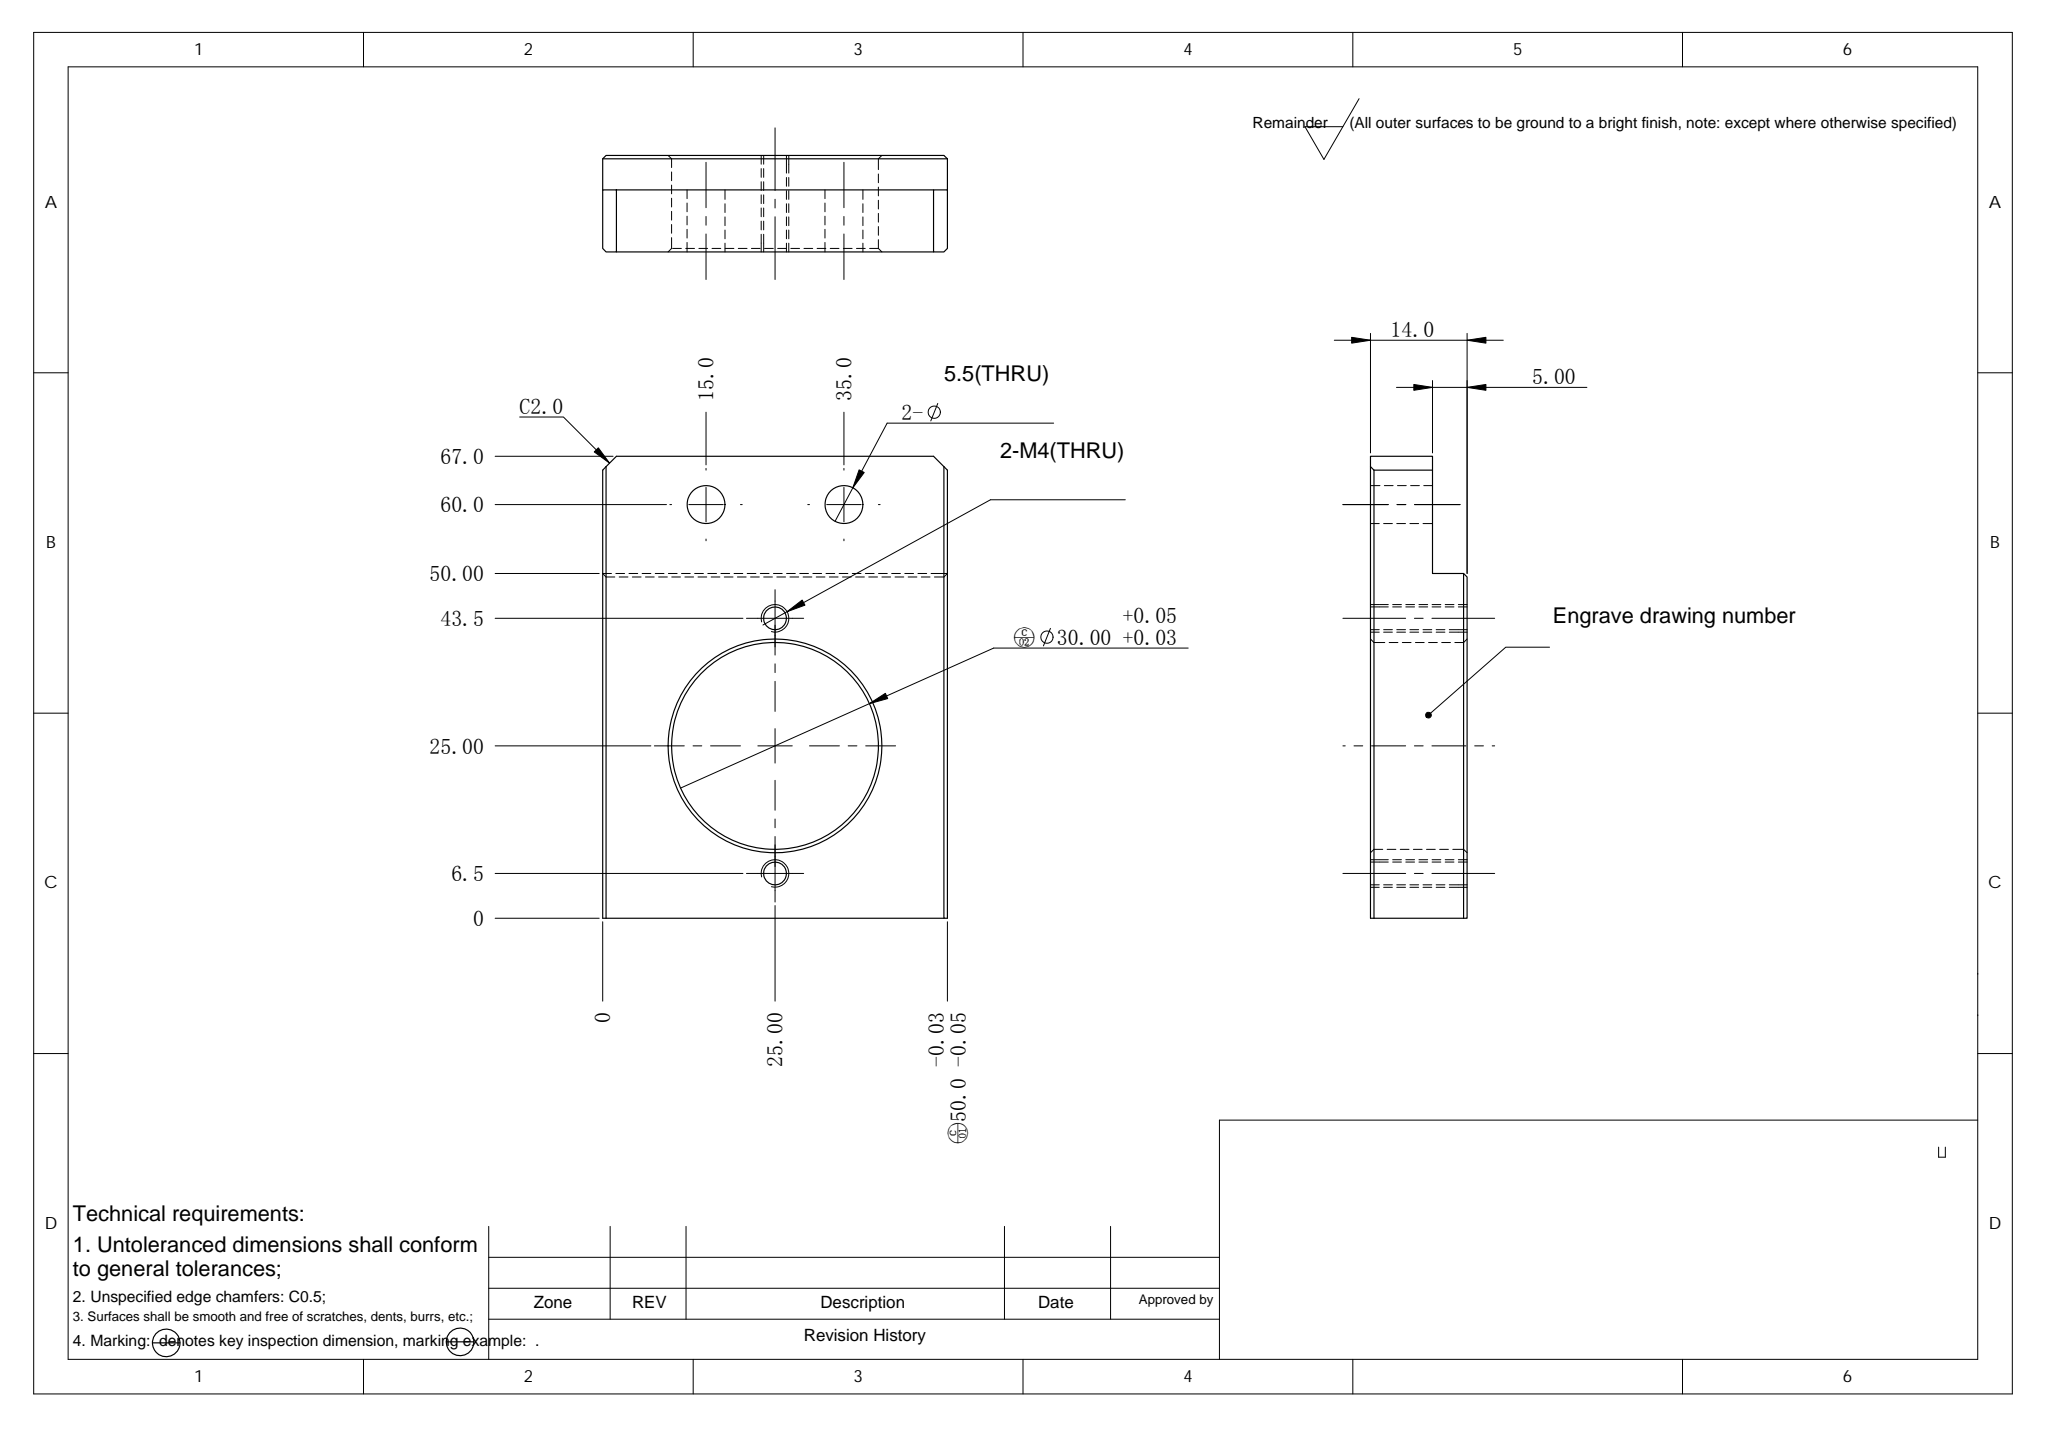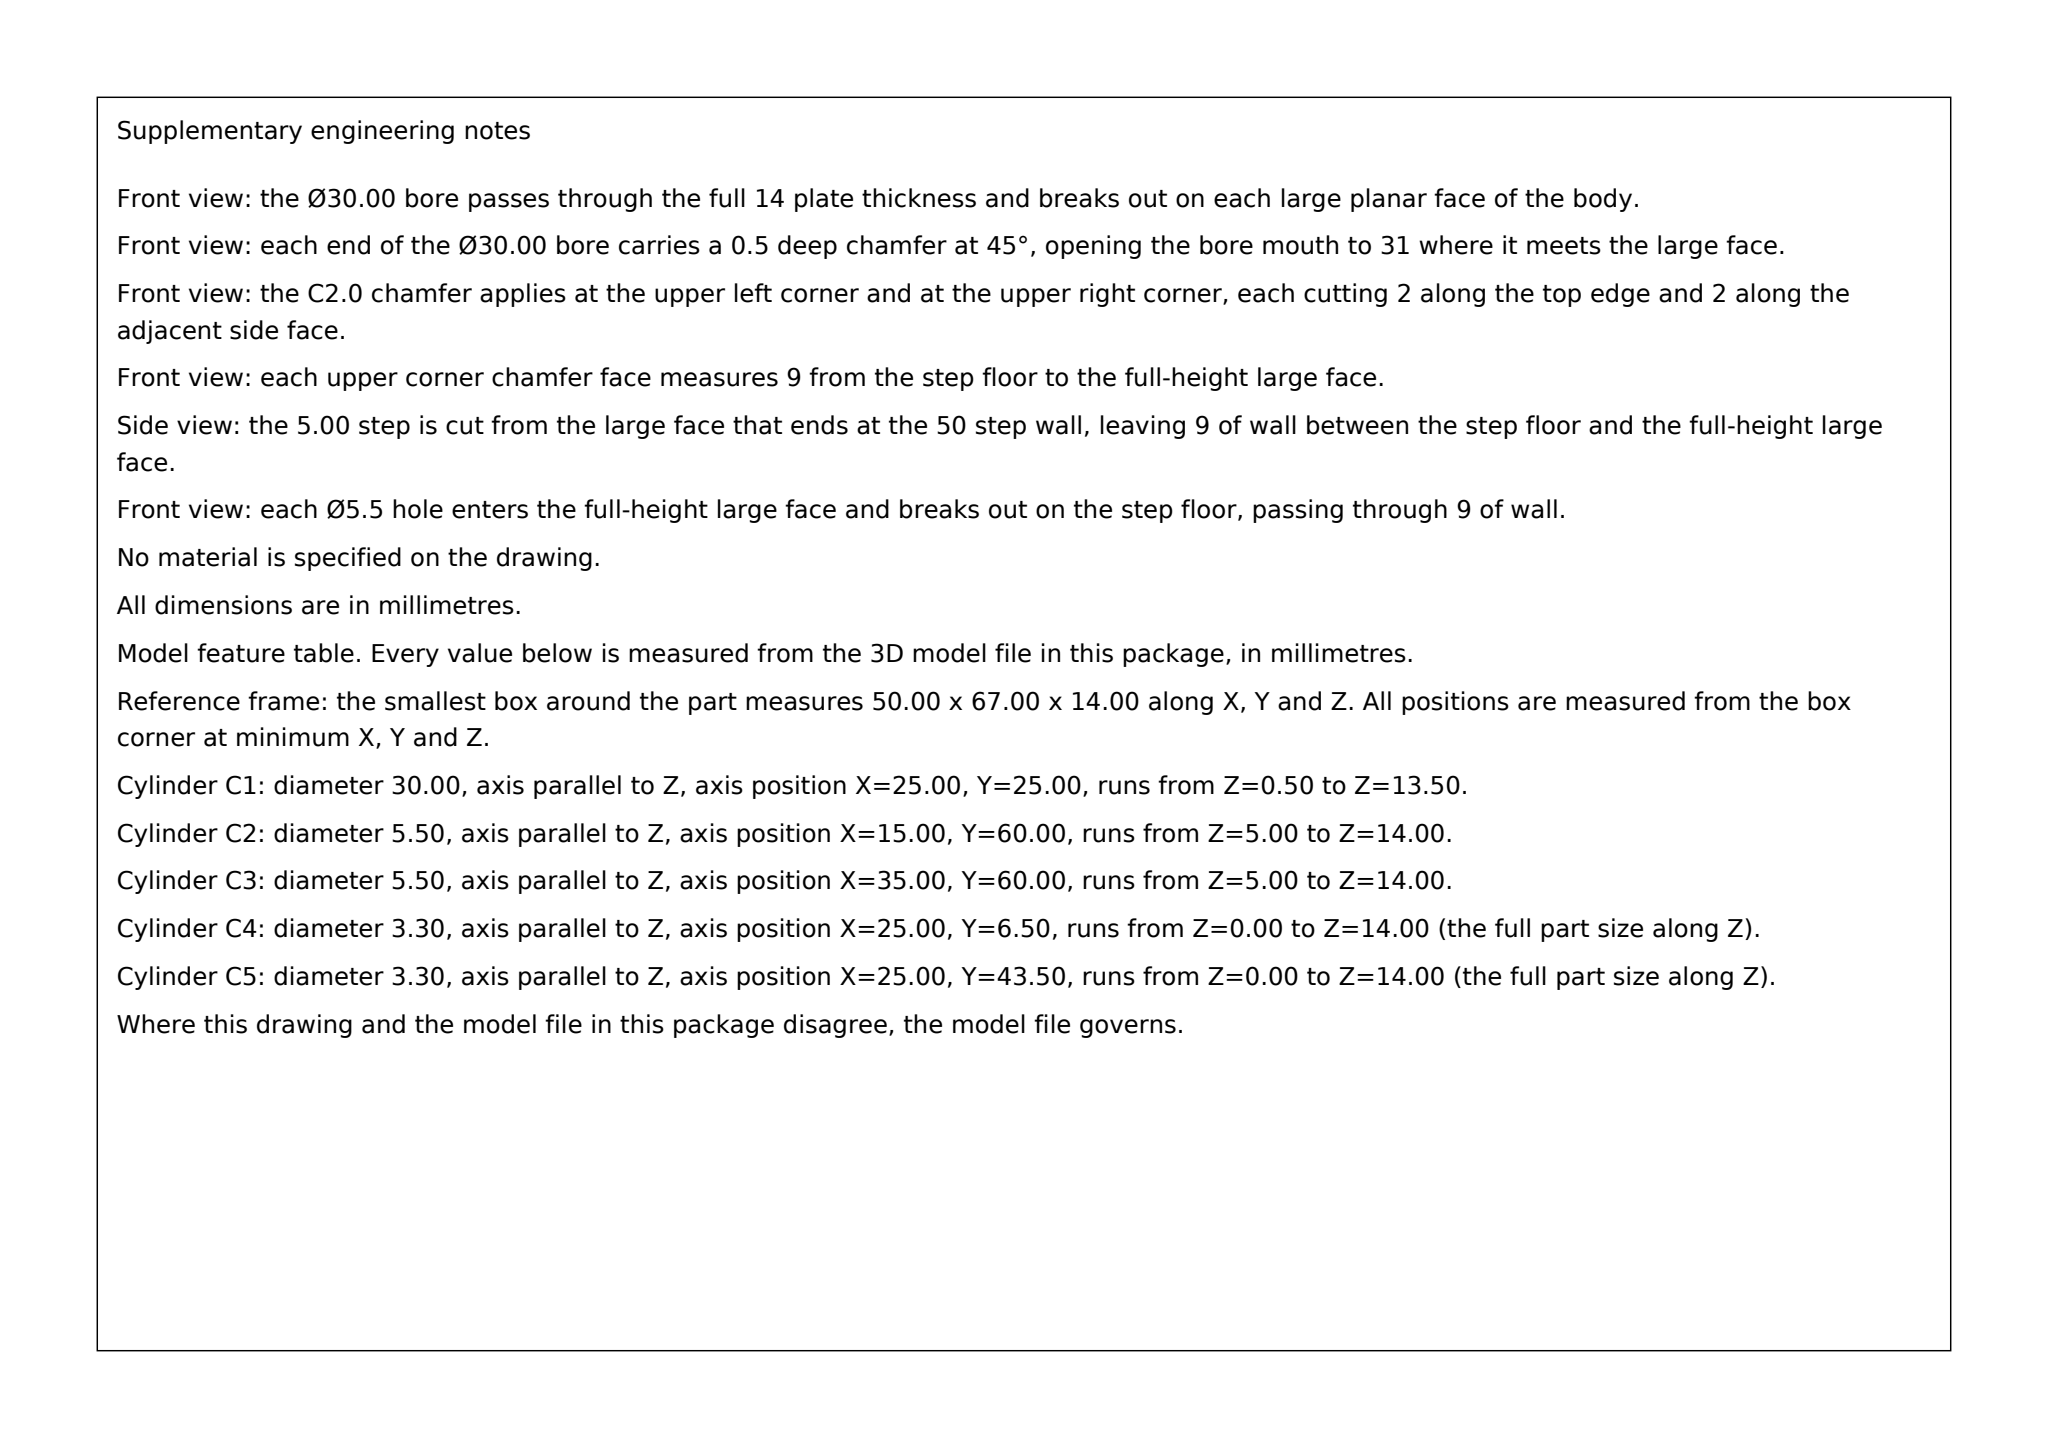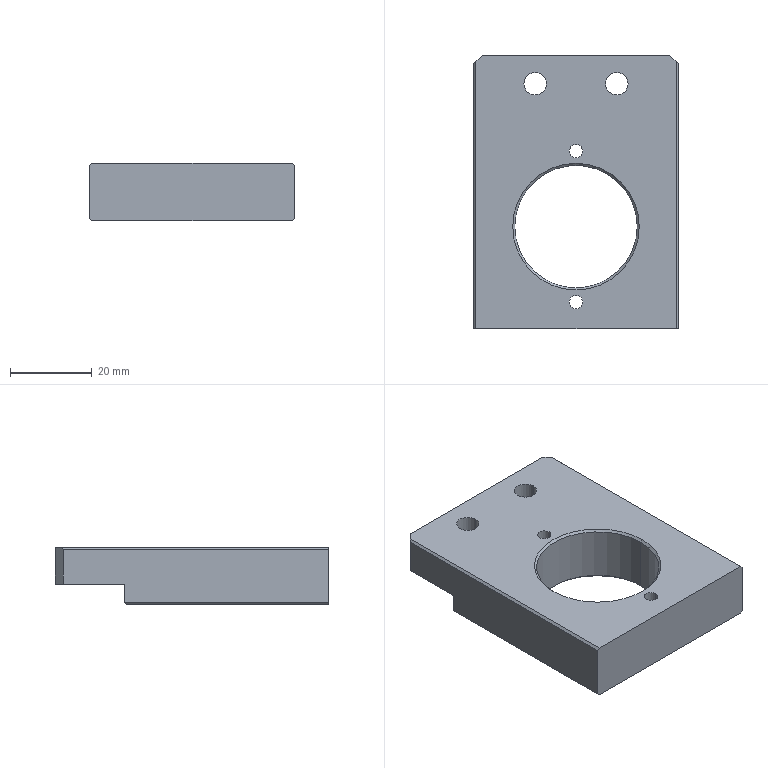Part | SolidWorks | mm | 1 solid | 29 faces | box 50 x 67 x 14 mm | volume 31992 mm3 | plane 15 | cylinder 10 | cone 4 | commonest cylinder face diameters 3.3 x4 5.5 x4 30 x2
Drawing notes:
STEP 17.0 WIDE (Y50.0-67.0) x FULL 50.0 x 5.00 DP | from the solid: z plane 5.0 step; y planes 50.0 and 67.0; x extent 0 to 50.0
Ø30.00 BORE THRU 14.0 THK | from the solid: Ø30 cyl L=13.0 + 0.5 chamfer each end = 14.0 = part thickness (z planes 0 and 14.0)
Ø30.00 BORE: C0.5 x 45° BOTH ENDS (TO Ø31.0) | from the solid: cones 90° incl, ref dia 30.0 to 31.0, qty 2 (one each end of bore)
2X C2.0 x 45° CHAMFER ON TOP CORNERS (AT Y=67.0, X=0 AND X=50.0), FULL DEPTH FROM Z=5.0 TO Z=14.0 | from the solid: inclined_planes: angle_to_xyz_axes [45,45,90] at bbox_from [0,65,5] and [48,65,5], size [2,2,9]
build123d program:
from build123d import *

# Parameters (mm, degrees)
SKETCH1_W                      = 50
SKETCH1_H                      = 70
BOSS_EXTRUDE1_DEPTH            = 14
SKETCH2_W                      = 5
SKETCH2_H                      = 20
CUT_EXTRUDE1_DEPTH             = 88.155
SKETCH3_R                      = 15
CUT_EXTRUDE2_DEPTH             = 88.155
F_5_5_5_5_DIAMETER_HOLE1_D     = 5.5
F_5_5_5_5_DIAMETER_HOLE1_DEPTH = 12
F_5_5_5_5_DIAMETER_HOLE1_TIP   = 1.652
M4_TAPPED_HOLE1_D              = 3.3
CHAMFER2_SIZE                  = 0.5
SKETCH8_W                      = 50
SKETCH8_H                      = 3
CUT_EXTRUDE3_DEPTH             = 88.155
CHAMFER3_SIZE                  = 2


with BuildPart() as part:
    # Sketch1 → Boss-Extrude1 (new body)
    with BuildSketch(Plane.XY):
        with Locations((25, 35)):
            Rectangle(SKETCH1_W, SKETCH1_H)
    extrude(amount=BOSS_EXTRUDE1_DEPTH)

    # Sketch2 → Cut-Extrude1 (cut, through all)
    with BuildSketch(Plane(origin=(50, 0, 0), x_dir=(0, 0, -1), z_dir=(1, 0, 0))):
        with Locations((-2.5, 60)):
            Rectangle(SKETCH2_W, SKETCH2_H)
    extrude(amount=-CUT_EXTRUDE1_DEPTH, mode=Mode.SUBTRACT)

    # Sketch3 → Cut-Extrude2 (cut, through all)
    with BuildSketch(Plane.XY.offset(14)):
        with Locations((25, 25)):
            Circle(SKETCH3_R)
    extrude(amount=-CUT_EXTRUDE2_DEPTH, mode=Mode.SUBTRACT)

    # 5.5 _5.5_ Diameter Hole1
    with Locations(Plane.XY.offset(14)):
        with Locations((15, 60), (35, 60)):
            Hole(F_5_5_5_5_DIAMETER_HOLE1_D / 2, depth=F_5_5_5_5_DIAMETER_HOLE1_DEPTH)
            with Locations((0, 0, -(F_5_5_5_5_DIAMETER_HOLE1_DEPTH + F_5_5_5_5_DIAMETER_HOLE1_TIP / 2))):  # 118° drill point
                Cone(0, F_5_5_5_5_DIAMETER_HOLE1_D / 2, F_5_5_5_5_DIAMETER_HOLE1_TIP, mode=Mode.SUBTRACT)

    # M4 Tapped Hole1 (through all)
    with Locations(Plane.XY.offset(14)):
        with Locations((25, 43.5), (25, 6.5)):
            Hole(M4_TAPPED_HOLE1_D / 2)

    # Chamfer2
    chamfer2_edges = [part.edges().sort_by_distance(p)[0] for p in [
        (50, 35, 14),
        (0, 25, 0),
        (25, 50, 0),
        (10, 25, 0),
        (10, 25, 14),
        (0, 35, 14),
        (50, 25, 0),
    ]]
    chamfer(chamfer2_edges, length=CHAMFER2_SIZE)

    # Sketch8 → Cut-Extrude3 (cut, through all)
    with BuildSketch(Plane.XY.offset(14)):
        with Locations((25, 68.5)):
            Rectangle(SKETCH8_W, SKETCH8_H)
    extrude(amount=-CUT_EXTRUDE3_DEPTH, mode=Mode.SUBTRACT)

    # Chamfer3
    chamfer3_edges = [part.edges().sort_by_distance(p)[0] for p in [
        (0, 67, 9.25),
        (50, 67, 9.25),
    ]]
    chamfer(chamfer3_edges, length=CHAMFER3_SIZE)


solid = part.part
STEP:
#1=CARTESIAN_POINT('',(10.,25.,13.5));
#2=VERTEX_POINT('',#1);
#3=CARTESIAN_POINT('',(40.,25.,13.5));
#4=VERTEX_POINT('',#3);
#5=CARTESIAN_POINT('',(25.,25.,13.5));
#6=DIRECTION('',(0.,0.,1.));
#7=DIRECTION('',(-1.,0.,0.));
#8=AXIS2_PLACEMENT_3D('',#5,#6,#7);
#9=CIRCLE('',#8,15.);
#10=EDGE_CURVE('',#2,#4,#9,.T.);
#11=ORIENTED_EDGE('',*,*,#10,.F.);
#12=CARTESIAN_POINT('',(9.5,25.,14.));
#13=VERTEX_POINT('',#12);
#14=CARTESIAN_POINT('',(10.,25.,13.5));
#15=DIRECTION('',(-0.7071,0.,0.7071));
#16=VECTOR('',#15,1000.);
#17=LINE('',#14,#16);
#18=EDGE_CURVE('',#2,#13,#17,.T.);
#19=ORIENTED_EDGE('',*,*,#18,.T.);
#20=CARTESIAN_POINT('',(40.5,25.,14.));
#21=VERTEX_POINT('',#20);
#22=CARTESIAN_POINT('',(25.,25.,14.));
#23=DIRECTION('',(0.,0.,-1.));
#24=DIRECTION('',(-1.,0.,0.));
#25=AXIS2_PLACEMENT_3D('',#22,#23,#24);
#26=CIRCLE('',#25,15.5);
#27=EDGE_CURVE('',#21,#13,#26,.T.);
#28=ORIENTED_EDGE('',*,*,#27,.F.);
#29=CARTESIAN_POINT('',(40.,25.,13.5));
#30=DIRECTION('',(0.7071,0.,0.7071));
#31=VECTOR('',#30,1000.);
#32=LINE('',#29,#31);
#33=EDGE_CURVE('',#4,#21,#32,.T.);
#34=ORIENTED_EDGE('',*,*,#33,.F.);
#35=EDGE_LOOP('',(#11,#19,#28,#34));
#36=FACE_OUTER_BOUND('',#35,.T.);
#37=CARTESIAN_POINT('',(25.,25.,13.5));
#38=DIRECTION('',(0.,0.,1.));
#39=DIRECTION('',(1.,0.,0.));
#40=AXIS2_PLACEMENT_3D('',#37,#38,#39);
#41=CONICAL_SURFACE('',#40,15.,0.7854);
#42=ADVANCED_FACE('',(#36),#41,.F.);
#43=CARTESIAN_POINT('',(40.,25.,0.5));
#44=VERTEX_POINT('',#43);
#45=CARTESIAN_POINT('',(10.,25.,0.5));
#46=VERTEX_POINT('',#45);
#47=CARTESIAN_POINT('',(25.,25.,0.5));
#48=DIRECTION('',(0.,0.,-1.));
#49=DIRECTION('',(-1.,0.,0.));
#50=AXIS2_PLACEMENT_3D('',#47,#48,#49);
#51=CIRCLE('',#50,15.);
#52=EDGE_CURVE('',#44,#46,#51,.T.);
#53=ORIENTED_EDGE('',*,*,#52,.F.);
#54=CARTESIAN_POINT('',(40.5,25.,0.));
#55=VERTEX_POINT('',#54);
#56=CARTESIAN_POINT('',(40.5,25.,0.));
#57=DIRECTION('',(0.7071,0.,-0.7071));
#58=VECTOR('',#57,1000.);
#59=LINE('',#56,#58);
#60=EDGE_CURVE('',#44,#55,#59,.T.);
#61=ORIENTED_EDGE('',*,*,#60,.T.);
#62=CARTESIAN_POINT('',(9.5,25.,0.));
#63=VERTEX_POINT('',#62);
#64=CARTESIAN_POINT('',(25.,25.,0.));
#65=DIRECTION('',(0.,0.,1.));
#66=DIRECTION('',(-1.,0.,0.));
#67=AXIS2_PLACEMENT_3D('',#64,#65,#66);
#68=CIRCLE('',#67,15.5);
#69=EDGE_CURVE('',#63,#55,#68,.T.);
#70=ORIENTED_EDGE('',*,*,#69,.F.);
#71=CARTESIAN_POINT('',(9.5,25.,0.));
#72=DIRECTION('',(-0.7071,0.,-0.7071));
#73=VECTOR('',#72,1000.);
#74=LINE('',#71,#73);
#75=EDGE_CURVE('',#46,#63,#74,.T.);
#76=ORIENTED_EDGE('',*,*,#75,.F.);
#77=EDGE_LOOP('',(#53,#61,#70,#76));
#78=FACE_OUTER_BOUND('',#77,.T.);
#79=CARTESIAN_POINT('',(25.,25.,0.));
#80=DIRECTION('',(0.,0.,-1.));
#81=DIRECTION('',(-1.,0.,0.));
#82=AXIS2_PLACEMENT_3D('',#79,#80,#81);
#83=CONICAL_SURFACE('',#82,15.5,0.7854);
#84=ADVANCED_FACE('',(#78),#83,.F.);
#85=CARTESIAN_POINT('',(23.35,43.5,-0.));
#86=VERTEX_POINT('',#85);
#87=CARTESIAN_POINT('',(26.65,43.5,-0.));
#88=VERTEX_POINT('',#87);
#89=CARTESIAN_POINT('',(25.,43.5,-0.));
#90=DIRECTION('',(0.,0.,1.));
#91=DIRECTION('',(1.,0.,0.));
#92=AXIS2_PLACEMENT_3D('',#89,#90,#91);
#93=CIRCLE('',#92,1.65);
#94=EDGE_CURVE('',#86,#88,#93,.T.);
#95=ORIENTED_EDGE('',*,*,#94,.F.);
#96=CARTESIAN_POINT('',(23.35,43.5,14.));
#97=VERTEX_POINT('',#96);
#98=CARTESIAN_POINT('',(23.35,43.5,14.));
#99=DIRECTION('',(0.,0.,1.));
#100=VECTOR('',#99,1000.);
#101=LINE('',#98,#100);
#102=EDGE_CURVE('',#86,#97,#101,.T.);
#103=ORIENTED_EDGE('',*,*,#102,.T.);
#104=CARTESIAN_POINT('',(26.65,43.5,14.));
#105=VERTEX_POINT('',#104);
#106=CARTESIAN_POINT('',(25.,43.5,14.));
#107=DIRECTION('',(0.,0.,1.));
#108=DIRECTION('',(1.,0.,0.));
#109=AXIS2_PLACEMENT_3D('',#106,#107,#108);
#110=CIRCLE('',#109,1.65);
#111=EDGE_CURVE('',#97,#105,#110,.T.);
#112=ORIENTED_EDGE('',*,*,#111,.T.);
#113=CARTESIAN_POINT('',(26.65,43.5,14.));
#114=DIRECTION('',(0.,0.,1.));
#115=VECTOR('',#114,1000.);
#116=LINE('',#113,#115);
#117=EDGE_CURVE('',#88,#105,#116,.T.);
#118=ORIENTED_EDGE('',*,*,#117,.F.);
#119=EDGE_LOOP('',(#95,#103,#112,#118));
#120=FACE_OUTER_BOUND('',#119,.T.);
#121=CARTESIAN_POINT('',(25.,43.5,14.));
#122=DIRECTION('',(0.,0.,1.));
#123=DIRECTION('',(1.,0.,0.));
#124=AXIS2_PLACEMENT_3D('',#121,#122,#123);
#125=CYLINDRICAL_SURFACE('',#124,1.65);
#126=ADVANCED_FACE('',(#120),#125,.F.);
#127=CARTESIAN_POINT('',(23.35,6.5,-0.));
#128=VERTEX_POINT('',#127);
#129=CARTESIAN_POINT('',(26.65,6.5,-0.));
#130=VERTEX_POINT('',#129);
#131=CARTESIAN_POINT('',(25.,6.5,-0.));
#132=DIRECTION('',(0.,0.,1.));
#133=DIRECTION('',(1.,0.,0.));
#134=AXIS2_PLACEMENT_3D('',#131,#132,#133);
#135=CIRCLE('',#134,1.65);
#136=EDGE_CURVE('',#128,#130,#135,.T.);
#137=ORIENTED_EDGE('',*,*,#136,.F.);
#138=CARTESIAN_POINT('',(23.35,6.5,14.));
#139=VERTEX_POINT('',#138);
#140=CARTESIAN_POINT('',(23.35,6.5,14.));
#141=DIRECTION('',(0.,0.,1.));
#142=VECTOR('',#141,1000.);
#143=LINE('',#140,#142);
#144=EDGE_CURVE('',#128,#139,#143,.T.);
#145=ORIENTED_EDGE('',*,*,#144,.T.);
#146=CARTESIAN_POINT('',(26.65,6.5,14.));
#147=VERTEX_POINT('',#146);
#148=CARTESIAN_POINT('',(25.,6.5,14.));
#149=DIRECTION('',(0.,0.,1.));
#150=DIRECTION('',(1.,0.,0.));
#151=AXIS2_PLACEMENT_3D('',#148,#149,#150);
#152=CIRCLE('',#151,1.65);
#153=EDGE_CURVE('',#139,#147,#152,.T.);
#154=ORIENTED_EDGE('',*,*,#153,.T.);
#155=CARTESIAN_POINT('',(26.65,6.5,14.));
#156=DIRECTION('',(0.,0.,1.));
#157=VECTOR('',#156,1000.);
#158=LINE('',#155,#157);
#159=EDGE_CURVE('',#130,#147,#158,.T.);
#160=ORIENTED_EDGE('',*,*,#159,.F.);
#161=EDGE_LOOP('',(#137,#145,#154,#160));
#162=FACE_OUTER_BOUND('',#161,.T.);
#163=CARTESIAN_POINT('',(25.,6.5,14.));
#164=DIRECTION('',(0.,0.,1.));
#165=DIRECTION('',(1.,0.,0.));
#166=AXIS2_PLACEMENT_3D('',#163,#164,#165);
#167=CYLINDRICAL_SURFACE('',#166,1.65);
#168=ADVANCED_FACE('',(#162),#167,.F.);
#169=CARTESIAN_POINT('',(12.25,60.,5.));
#170=VERTEX_POINT('',#169);
#171=CARTESIAN_POINT('',(17.75,60.,5.));
#172=VERTEX_POINT('',#171);
#173=CARTESIAN_POINT('',(15.,60.,5.));
#174=DIRECTION('',(0.,-0.,1.));
#175=DIRECTION('',(0.,-1.,0.));
#176=AXIS2_PLACEMENT_3D('',#173,#174,#175);
#177=CIRCLE('',#176,2.75);
#178=EDGE_CURVE('',#170,#172,#177,.T.);
#179=ORIENTED_EDGE('',*,*,#178,.F.);
#180=CARTESIAN_POINT('',(12.25,60.,14.));
#181=VERTEX_POINT('',#180);
#182=CARTESIAN_POINT('',(12.25,60.,14.));
#183=DIRECTION('',(0.,0.,1.));
#184=VECTOR('',#183,1000.);
#185=LINE('',#182,#184);
#186=EDGE_CURVE('',#170,#181,#185,.T.);
#187=ORIENTED_EDGE('',*,*,#186,.T.);
#188=CARTESIAN_POINT('',(17.75,60.,14.));
#189=VERTEX_POINT('',#188);
#190=CARTESIAN_POINT('',(15.,60.,14.));
#191=DIRECTION('',(0.,0.,1.));
#192=DIRECTION('',(1.,0.,0.));
#193=AXIS2_PLACEMENT_3D('',#190,#191,#192);
#194=CIRCLE('',#193,2.75);
#195=EDGE_CURVE('',#181,#189,#194,.T.);
#196=ORIENTED_EDGE('',*,*,#195,.T.);
#197=CARTESIAN_POINT('',(17.75,60.,14.));
#198=DIRECTION('',(0.,0.,1.));
#199=VECTOR('',#198,1000.);
#200=LINE('',#197,#199);
#201=EDGE_CURVE('',#172,#189,#200,.T.);
#202=ORIENTED_EDGE('',*,*,#201,.F.);
#203=EDGE_LOOP('',(#179,#187,#196,#202));
#204=FACE_OUTER_BOUND('',#203,.T.);
#205=CARTESIAN_POINT('',(15.,60.,14.));
#206=DIRECTION('',(0.,0.,1.));
#207=DIRECTION('',(1.,0.,0.));
#208=AXIS2_PLACEMENT_3D('',#205,#206,#207);
#209=CYLINDRICAL_SURFACE('',#208,2.75);
#210=ADVANCED_FACE('',(#204),#209,.F.);
#211=CARTESIAN_POINT('',(32.25,60.,5.));
#212=VERTEX_POINT('',#211);
#213=CARTESIAN_POINT('',(37.75,60.,5.));
#214=VERTEX_POINT('',#213);
#215=CARTESIAN_POINT('',(35.,60.,5.));
#216=DIRECTION('',(0.,-0.,1.));
#217=DIRECTION('',(0.,-1.,0.));
#218=AXIS2_PLACEMENT_3D('',#215,#216,#217);
#219=CIRCLE('',#218,2.75);
#220=EDGE_CURVE('',#212,#214,#219,.T.);
#221=ORIENTED_EDGE('',*,*,#220,.F.);
#222=CARTESIAN_POINT('',(32.25,60.,14.));
#223=VERTEX_POINT('',#222);
#224=CARTESIAN_POINT('',(32.25,60.,14.));
#225=DIRECTION('',(0.,0.,1.));
#226=VECTOR('',#225,1000.);
#227=LINE('',#224,#226);
#228=EDGE_CURVE('',#212,#223,#227,.T.);
#229=ORIENTED_EDGE('',*,*,#228,.T.);
#230=CARTESIAN_POINT('',(37.75,60.,14.));
#231=VERTEX_POINT('',#230);
#232=CARTESIAN_POINT('',(35.,60.,14.));
#233=DIRECTION('',(0.,0.,1.));
#234=DIRECTION('',(1.,0.,0.));
#235=AXIS2_PLACEMENT_3D('',#232,#233,#234);
#236=CIRCLE('',#235,2.75);
#237=EDGE_CURVE('',#223,#231,#236,.T.);
#238=ORIENTED_EDGE('',*,*,#237,.T.);
#239=CARTESIAN_POINT('',(37.75,60.,14.));
#240=DIRECTION('',(0.,0.,1.));
#241=VECTOR('',#240,1000.);
#242=LINE('',#239,#241);
#243=EDGE_CURVE('',#214,#231,#242,.T.);
#244=ORIENTED_EDGE('',*,*,#243,.F.);
#245=EDGE_LOOP('',(#221,#229,#238,#244));
#246=FACE_OUTER_BOUND('',#245,.T.);
#247=CARTESIAN_POINT('',(35.,60.,14.));
#248=DIRECTION('',(0.,0.,1.));
#249=DIRECTION('',(1.,0.,0.));
#250=AXIS2_PLACEMENT_3D('',#247,#248,#249);
#251=CYLINDRICAL_SURFACE('',#250,2.75);
#252=ADVANCED_FACE('',(#246),#251,.F.);
#253=ORIENTED_EDGE('',*,*,#52,.T.);
#254=CARTESIAN_POINT('',(10.,25.,-0.));
#255=DIRECTION('',(0.,0.,1.));
#256=VECTOR('',#255,1000.);
#257=LINE('',#254,#256);
#258=EDGE_CURVE('',#46,#2,#257,.T.);
#259=ORIENTED_EDGE('',*,*,#258,.T.);
#260=ORIENTED_EDGE('',*,*,#10,.T.);
#261=CARTESIAN_POINT('',(40.,25.,-0.));
#262=DIRECTION('',(0.,0.,1.));
#263=VECTOR('',#262,1000.);
#264=LINE('',#261,#263);
#265=EDGE_CURVE('',#44,#4,#264,.T.);
#266=ORIENTED_EDGE('',*,*,#265,.F.);
#267=EDGE_LOOP('',(#253,#259,#260,#266));
#268=FACE_OUTER_BOUND('',#267,.T.);
#269=CARTESIAN_POINT('',(25.,25.,-0.));
#270=DIRECTION('',(0.,0.,1.));
#271=DIRECTION('',(1.,0.,0.));
#272=AXIS2_PLACEMENT_3D('',#269,#270,#271);
#273=CYLINDRICAL_SURFACE('',#272,15.);
#274=ADVANCED_FACE('',(#268),#273,.F.);
#275=CARTESIAN_POINT('',(0.,0.,13.5));
#276=VERTEX_POINT('',#275);
#277=CARTESIAN_POINT('',(0.,65.,13.5));
#278=VERTEX_POINT('',#277);
#279=CARTESIAN_POINT('',(0.,0.,13.5));
#280=DIRECTION('',(0.,1.,0.));
#281=VECTOR('',#280,1000.);
#282=LINE('',#279,#281);
#283=EDGE_CURVE('',#276,#278,#282,.T.);
#284=ORIENTED_EDGE('',*,*,#283,.T.);
#285=CARTESIAN_POINT('',(-0.,65.,5.));
#286=VERTEX_POINT('',#285);
#287=CARTESIAN_POINT('',(0.,65.,14.));
#288=DIRECTION('',(0.,0.,-1.));
#289=VECTOR('',#288,1000.);
#290=LINE('',#287,#289);
#291=EDGE_CURVE('',#278,#286,#290,.T.);
#292=ORIENTED_EDGE('',*,*,#291,.T.);
#293=CARTESIAN_POINT('',(0.,50.,5.));
#294=VERTEX_POINT('',#293);
#295=CARTESIAN_POINT('',(0.,70.,5.));
#296=DIRECTION('',(0.,-1.,-0.));
#297=VECTOR('',#296,1000.);
#298=LINE('',#295,#297);
#299=EDGE_CURVE('',#286,#294,#298,.T.);
#300=ORIENTED_EDGE('',*,*,#299,.T.);
#301=CARTESIAN_POINT('',(0.,50.,0.5));
#302=VERTEX_POINT('',#301);
#303=CARTESIAN_POINT('',(0.,50.,-0.));
#304=DIRECTION('',(0.,0.,-1.));
#305=VECTOR('',#304,1000.);
#306=LINE('',#303,#305);
#307=EDGE_CURVE('',#294,#302,#306,.T.);
#308=ORIENTED_EDGE('',*,*,#307,.T.);
#309=CARTESIAN_POINT('',(-0.,0.,0.5));
#310=VERTEX_POINT('',#309);
#311=CARTESIAN_POINT('',(0.,0.,0.5));
#312=DIRECTION('',(0.,-1.,0.));
#313=VECTOR('',#312,1000.);
#314=LINE('',#311,#313);
#315=EDGE_CURVE('',#302,#310,#314,.T.);
#316=ORIENTED_EDGE('',*,*,#315,.T.);
#317=CARTESIAN_POINT('',(0.,0.,14.));
#318=DIRECTION('',(0.,0.,-1.));
#319=VECTOR('',#318,1000.);
#320=LINE('',#317,#319);
#321=EDGE_CURVE('',#276,#310,#320,.T.);
#322=ORIENTED_EDGE('',*,*,#321,.F.);
#323=EDGE_LOOP('',(#284,#292,#300,#308,#316,#322));
#324=FACE_OUTER_BOUND('',#323,.T.);
#325=CARTESIAN_POINT('',(0.,0.,14.));
#326=DIRECTION('',(1.,0.,0.));
#327=DIRECTION('',(0.,0.,-1.));
#328=AXIS2_PLACEMENT_3D('',#325,#326,#327);
#329=PLANE('',#328);
#330=ADVANCED_FACE('',(#324),#329,.F.);
#331=CARTESIAN_POINT('',(0.5,0.,14.));
#332=VERTEX_POINT('',#331);
#333=CARTESIAN_POINT('',(49.5,0.,14.));
#334=VERTEX_POINT('',#333);
#335=CARTESIAN_POINT('',(0.,0.,14.));
#336=DIRECTION('',(1.,0.,0.));
#337=VECTOR('',#336,1000.);
#338=LINE('',#335,#337);
#339=EDGE_CURVE('',#332,#334,#338,.T.);
#340=ORIENTED_EDGE('',*,*,#339,.F.);
#341=CARTESIAN_POINT('',(0.5,0.,14.));
#342=DIRECTION('',(-0.7071,0.,-0.7071));
#343=VECTOR('',#342,1000.);
#344=LINE('',#341,#343);
#345=EDGE_CURVE('',#332,#276,#344,.T.);
#346=ORIENTED_EDGE('',*,*,#345,.T.);
#347=ORIENTED_EDGE('',*,*,#321,.T.);
#348=CARTESIAN_POINT('',(0.5,0.,0.));
#349=VERTEX_POINT('',#348);
#350=CARTESIAN_POINT('',(0.,0.,0.5));
#351=DIRECTION('',(0.7071,0.,-0.7071));
#352=VECTOR('',#351,1000.);
#353=LINE('',#350,#352);
#354=EDGE_CURVE('',#310,#349,#353,.T.);
#355=ORIENTED_EDGE('',*,*,#354,.T.);
#356=CARTESIAN_POINT('',(49.5,0.,-0.));
#357=VERTEX_POINT('',#356);
#358=CARTESIAN_POINT('',(0.,0.,0.));
#359=DIRECTION('',(1.,0.,0.));
#360=VECTOR('',#359,1000.);
#361=LINE('',#358,#360);
#362=EDGE_CURVE('',#349,#357,#361,.T.);
#363=ORIENTED_EDGE('',*,*,#362,.T.);
#364=CARTESIAN_POINT('',(50.,0.,0.5));
#365=VERTEX_POINT('',#364);
#366=CARTESIAN_POINT('',(50.,0.,0.5));
#367=DIRECTION('',(0.7071,0.,0.7071));
#368=VECTOR('',#367,1000.);
#369=LINE('',#366,#368);
#370=EDGE_CURVE('',#357,#365,#369,.T.);
#371=ORIENTED_EDGE('',*,*,#370,.T.);
#372=CARTESIAN_POINT('',(50.,0.,13.5));
#373=VERTEX_POINT('',#372);
#374=CARTESIAN_POINT('',(50.,0.,14.));
#375=DIRECTION('',(0.,0.,-1.));
#376=VECTOR('',#375,1000.);
#377=LINE('',#374,#376);
#378=EDGE_CURVE('',#373,#365,#377,.T.);
#379=ORIENTED_EDGE('',*,*,#378,.F.);
#380=CARTESIAN_POINT('',(49.5,0.,14.));
#381=DIRECTION('',(-0.7071,0.,0.7071));
#382=VECTOR('',#381,1000.);
#383=LINE('',#380,#382);
#384=EDGE_CURVE('',#373,#334,#383,.T.);
#385=ORIENTED_EDGE('',*,*,#384,.T.);
#386=EDGE_LOOP('',(#340,#346,#347,#355,#363,#371,#379,#385));
#387=FACE_OUTER_BOUND('',#386,.T.);
#388=CARTESIAN_POINT('',(0.,0.,14.));
#389=DIRECTION('',(0.,1.,0.));
#390=DIRECTION('',(0.,0.,1.));
#391=AXIS2_PLACEMENT_3D('',#388,#389,#390);
#392=PLANE('',#391);
#393=ADVANCED_FACE('',(#387),#392,.F.);
#394=CARTESIAN_POINT('',(50.,65.,5.));
#395=VERTEX_POINT('',#394);
#396=CARTESIAN_POINT('',(50.,50.,5.));
#397=VERTEX_POINT('',#396);
#398=CARTESIAN_POINT('',(50.,70.,5.));
#399=DIRECTION('',(0.,-1.,-0.));
#400=VECTOR('',#399,1000.);
#401=LINE('',#398,#400);
#402=EDGE_CURVE('',#395,#397,#401,.T.);
#403=ORIENTED_EDGE('',*,*,#402,.F.);
#404=CARTESIAN_POINT('',(50.,65.,13.5));
#405=VERTEX_POINT('',#404);
#406=CARTESIAN_POINT('',(50.,65.,14.));
#407=DIRECTION('',(0.,0.,1.));
#408=VECTOR('',#407,1000.);
#409=LINE('',#406,#408);
#410=EDGE_CURVE('',#395,#405,#409,.T.);
#411=ORIENTED_EDGE('',*,*,#410,.T.);
#412=CARTESIAN_POINT('',(50.,0.,13.5));
#413=DIRECTION('',(0.,-1.,0.));
#414=VECTOR('',#413,1000.);
#415=LINE('',#412,#414);
#416=EDGE_CURVE('',#405,#373,#415,.T.);
#417=ORIENTED_EDGE('',*,*,#416,.T.);
#418=ORIENTED_EDGE('',*,*,#378,.T.);
#419=CARTESIAN_POINT('',(50.,50.,0.5));
#420=VERTEX_POINT('',#419);
#421=CARTESIAN_POINT('',(50.,50.,0.5));
#422=DIRECTION('',(0.,1.,0.));
#423=VECTOR('',#422,1000.);
#424=LINE('',#421,#423);
#425=EDGE_CURVE('',#365,#420,#424,.T.);
#426=ORIENTED_EDGE('',*,*,#425,.T.);
#427=CARTESIAN_POINT('',(50.,50.,-0.));
#428=DIRECTION('',(0.,0.,-1.));
#429=VECTOR('',#428,1000.);
#430=LINE('',#427,#429);
#431=EDGE_CURVE('',#397,#420,#430,.T.);
#432=ORIENTED_EDGE('',*,*,#431,.F.);
#433=EDGE_LOOP('',(#403,#411,#417,#418,#426,#432));
#434=FACE_OUTER_BOUND('',#433,.T.);
#435=CARTESIAN_POINT('',(50.,0.,14.));
#436=DIRECTION('',(-1.,0.,0.));
#437=DIRECTION('',(0.,0.,1.));
#438=AXIS2_PLACEMENT_3D('',#435,#436,#437);
#439=PLANE('',#438);
#440=ADVANCED_FACE('',(#434),#439,.F.);
#441=ORIENTED_EDGE('',*,*,#27,.T.);
#442=CARTESIAN_POINT('',(25.,25.,14.));
#443=DIRECTION('',(0.,0.,-1.));
#444=DIRECTION('',(-1.,0.,0.));
#445=AXIS2_PLACEMENT_3D('',#442,#443,#444);
#446=CIRCLE('',#445,15.5);
#447=EDGE_CURVE('',#13,#21,#446,.T.);
#448=ORIENTED_EDGE('',*,*,#447,.T.);
#449=EDGE_LOOP('',(#441,#448));
#450=FACE_BOUND('',#449,.T.);
#451=CARTESIAN_POINT('',(25.,43.5,14.));
#452=DIRECTION('',(0.,0.,1.));
#453=DIRECTION('',(1.,0.,0.));
#454=AXIS2_PLACEMENT_3D('',#451,#452,#453);
#455=CIRCLE('',#454,1.65);
#456=EDGE_CURVE('',#105,#97,#455,.T.);
#457=ORIENTED_EDGE('',*,*,#456,.F.);
#458=ORIENTED_EDGE('',*,*,#111,.F.);
#459=EDGE_LOOP('',(#457,#458));
#460=FACE_BOUND('',#459,.T.);
#461=CARTESIAN_POINT('',(25.,6.5,14.));
#462=DIRECTION('',(0.,0.,1.));
#463=DIRECTION('',(1.,0.,0.));
#464=AXIS2_PLACEMENT_3D('',#461,#462,#463);
#465=CIRCLE('',#464,1.65);
#466=EDGE_CURVE('',#147,#139,#465,.T.);
#467=ORIENTED_EDGE('',*,*,#466,.F.);
#468=ORIENTED_EDGE('',*,*,#153,.F.);
#469=EDGE_LOOP('',(#467,#468));
#470=FACE_BOUND('',#469,.T.);
#471=CARTESIAN_POINT('',(15.,60.,14.));
#472=DIRECTION('',(0.,0.,1.));
#473=DIRECTION('',(1.,0.,0.));
#474=AXIS2_PLACEMENT_3D('',#471,#472,#473);
#475=CIRCLE('',#474,2.75);
#476=EDGE_CURVE('',#189,#181,#475,.T.);
#477=ORIENTED_EDGE('',*,*,#476,.F.);
#478=ORIENTED_EDGE('',*,*,#195,.F.);
#479=EDGE_LOOP('',(#477,#478));
#480=FACE_BOUND('',#479,.T.);
#481=CARTESIAN_POINT('',(35.,60.,14.));
#482=DIRECTION('',(0.,0.,1.));
#483=DIRECTION('',(1.,0.,0.));
#484=AXIS2_PLACEMENT_3D('',#481,#482,#483);
#485=CIRCLE('',#484,2.75);
#486=EDGE_CURVE('',#231,#223,#485,.T.);
#487=ORIENTED_EDGE('',*,*,#486,.F.);
#488=ORIENTED_EDGE('',*,*,#237,.F.);
#489=EDGE_LOOP('',(#487,#488));
#490=FACE_BOUND('',#489,.T.);
#491=CARTESIAN_POINT('',(2.,67.,14.));
#492=VERTEX_POINT('',#491);
#493=CARTESIAN_POINT('',(48.,67.,14.));
#494=VERTEX_POINT('',#493);
#495=CARTESIAN_POINT('',(0.,67.,14.));
#496=DIRECTION('',(1.,0.,0.));
#497=VECTOR('',#496,1000.);
#498=LINE('',#495,#497);
#499=EDGE_CURVE('',#492,#494,#498,.T.);
#500=ORIENTED_EDGE('',*,*,#499,.F.);
#501=CARTESIAN_POINT('',(0.5,65.5,14.));
#502=VERTEX_POINT('',#501);
#503=CARTESIAN_POINT('',(2.,67.,14.));
#504=DIRECTION('',(-0.7071,-0.7071,0.));
#505=VECTOR('',#504,1000.);
#506=LINE('',#503,#505);
#507=EDGE_CURVE('',#492,#502,#506,.T.);
#508=ORIENTED_EDGE('',*,*,#507,.T.);
#509=CARTESIAN_POINT('',(0.5,0.,14.));
#510=DIRECTION('',(0.,-1.,0.));
#511=VECTOR('',#510,1000.);
#512=LINE('',#509,#511);
#513=EDGE_CURVE('',#502,#332,#512,.T.);
#514=ORIENTED_EDGE('',*,*,#513,.T.);
#515=ORIENTED_EDGE('',*,*,#339,.T.);
#516=CARTESIAN_POINT('',(49.5,65.5,14.));
#517=VERTEX_POINT('',#516);
#518=CARTESIAN_POINT('',(49.5,0.,14.));
#519=DIRECTION('',(0.,1.,0.));
#520=VECTOR('',#519,1000.);
#521=LINE('',#518,#520);
#522=EDGE_CURVE('',#334,#517,#521,.T.);
#523=ORIENTED_EDGE('',*,*,#522,.T.);
#524=CARTESIAN_POINT('',(50.,65.,14.));
#525=DIRECTION('',(-0.7071,0.7071,0.));
#526=VECTOR('',#525,1000.);
#527=LINE('',#524,#526);
#528=EDGE_CURVE('',#517,#494,#527,.T.);
#529=ORIENTED_EDGE('',*,*,#528,.T.);
#530=EDGE_LOOP('',(#500,#508,#514,#515,#523,#529));
#531=FACE_OUTER_BOUND('',#530,.T.);
#532=CARTESIAN_POINT('',(0.,0.,14.));
#533=DIRECTION('',(0.,0.,-1.));
#534=DIRECTION('',(-1.,0.,0.));
#535=AXIS2_PLACEMENT_3D('',#532,#533,#534);
#536=PLANE('',#535);
#537=ADVANCED_FACE('',(#450,#460,#470,#480,#490,#531),#536,.F.);
#538=ORIENTED_EDGE('',*,*,#69,.T.);
#539=CARTESIAN_POINT('',(25.,25.,0.));
#540=DIRECTION('',(0.,0.,1.));
#541=DIRECTION('',(-1.,0.,0.));
#542=AXIS2_PLACEMENT_3D('',#539,#540,#541);
#543=CIRCLE('',#542,15.5);
#544=EDGE_CURVE('',#55,#63,#543,.T.);
#545=ORIENTED_EDGE('',*,*,#544,.T.);
#546=EDGE_LOOP('',(#538,#545));
#547=FACE_BOUND('',#546,.T.);
#548=CARTESIAN_POINT('',(25.,43.5,-0.));
#549=DIRECTION('',(0.,0.,1.));
#550=DIRECTION('',(1.,0.,0.));
#551=AXIS2_PLACEMENT_3D('',#548,#549,#550);
#552=CIRCLE('',#551,1.65);
#553=EDGE_CURVE('',#88,#86,#552,.T.);
#554=ORIENTED_EDGE('',*,*,#553,.T.);
#555=ORIENTED_EDGE('',*,*,#94,.T.);
#556=EDGE_LOOP('',(#554,#555));
#557=FACE_BOUND('',#556,.T.);
#558=CARTESIAN_POINT('',(25.,6.5,-0.));
#559=DIRECTION('',(0.,0.,1.));
#560=DIRECTION('',(1.,0.,0.));
#561=AXIS2_PLACEMENT_3D('',#558,#559,#560);
#562=CIRCLE('',#561,1.65);
#563=EDGE_CURVE('',#130,#128,#562,.T.);
#564=ORIENTED_EDGE('',*,*,#563,.T.);
#565=ORIENTED_EDGE('',*,*,#136,.T.);
#566=EDGE_LOOP('',(#564,#565));
#567=FACE_BOUND('',#566,.T.);
#568=ORIENTED_EDGE('',*,*,#362,.F.);
#569=CARTESIAN_POINT('',(0.5,49.5,0.));
#570=VERTEX_POINT('',#569);
#571=CARTESIAN_POINT('',(0.5,50.,0.));
#572=DIRECTION('',(0.,1.,0.));
#573=VECTOR('',#572,1000.);
#574=LINE('',#571,#573);
#575=EDGE_CURVE('',#349,#570,#574,.T.);
#576=ORIENTED_EDGE('',*,*,#575,.T.);
#577=CARTESIAN_POINT('',(49.5,49.5,0.));
#578=VERTEX_POINT('',#577);
#579=CARTESIAN_POINT('',(50.,49.5,0.));
#580=DIRECTION('',(1.,0.,0.));
#581=VECTOR('',#580,1000.);
#582=LINE('',#579,#581);
#583=EDGE_CURVE('',#570,#578,#582,.T.);
#584=ORIENTED_EDGE('',*,*,#583,.T.);
#585=CARTESIAN_POINT('',(49.5,0.,0.));
#586=DIRECTION('',(0.,-1.,0.));
#587=VECTOR('',#586,1000.);
#588=LINE('',#585,#587);
#589=EDGE_CURVE('',#578,#357,#588,.T.);
#590=ORIENTED_EDGE('',*,*,#589,.T.);
#591=EDGE_LOOP('',(#568,#576,#584,#590));
#592=FACE_OUTER_BOUND('',#591,.T.);
#593=CARTESIAN_POINT('',(0.,0.,0.));
#594=DIRECTION('',(0.,0.,-1.));
#595=DIRECTION('',(-1.,0.,0.));
#596=AXIS2_PLACEMENT_3D('',#593,#594,#595);
#597=PLANE('',#596);
#598=ADVANCED_FACE('',(#547,#557,#567,#592),#597,.T.);
#599=ORIENTED_EDGE('',*,*,#431,.T.);
#600=CARTESIAN_POINT('',(0.,50.,0.5));
#601=DIRECTION('',(-1.,0.,0.));
#602=VECTOR('',#601,1000.);
#603=LINE('',#600,#602);
#604=EDGE_CURVE('',#420,#302,#603,.T.);
#605=ORIENTED_EDGE('',*,*,#604,.T.);
#606=ORIENTED_EDGE('',*,*,#307,.F.);
#607=CARTESIAN_POINT('',(0.,50.,5.));
#608=DIRECTION('',(1.,0.,0.));
#609=VECTOR('',#608,1000.);
#610=LINE('',#607,#609);
#611=EDGE_CURVE('',#294,#397,#610,.T.);
#612=ORIENTED_EDGE('',*,*,#611,.T.);
#613=EDGE_LOOP('',(#599,#605,#606,#612));
#614=FACE_OUTER_BOUND('',#613,.T.);
#615=CARTESIAN_POINT('',(0.,50.,-0.));
#616=DIRECTION('',(0.,-1.,0.));
#617=DIRECTION('',(0.,0.,-1.));
#618=AXIS2_PLACEMENT_3D('',#615,#616,#617);
#619=PLANE('',#618);
#620=ADVANCED_FACE('',(#614),#619,.F.);
#621=CARTESIAN_POINT('',(15.,60.,5.));
#622=DIRECTION('',(0.,-0.,1.));
#623=DIRECTION('',(0.,-1.,0.));
#624=AXIS2_PLACEMENT_3D('',#621,#622,#623);
#625=CIRCLE('',#624,2.75);
#626=EDGE_CURVE('',#172,#170,#625,.T.);
#627=ORIENTED_EDGE('',*,*,#626,.T.);
#628=ORIENTED_EDGE('',*,*,#178,.T.);
#629=EDGE_LOOP('',(#627,#628));
#630=FACE_BOUND('',#629,.T.);
#631=CARTESIAN_POINT('',(35.,60.,5.));
#632=DIRECTION('',(0.,-0.,1.));
#633=DIRECTION('',(0.,-1.,0.));
#634=AXIS2_PLACEMENT_3D('',#631,#632,#633);
#635=CIRCLE('',#634,2.75);
#636=EDGE_CURVE('',#214,#212,#635,.T.);
#637=ORIENTED_EDGE('',*,*,#636,.T.);
#638=ORIENTED_EDGE('',*,*,#220,.T.);
#639=EDGE_LOOP('',(#637,#638));
#640=FACE_BOUND('',#639,.T.);
#641=ORIENTED_EDGE('',*,*,#299,.F.);
#642=CARTESIAN_POINT('',(2.,67.,5.));
#643=VERTEX_POINT('',#642);
#644=CARTESIAN_POINT('',(2.,67.,5.));
#645=DIRECTION('',(0.7071,0.7071,0.));
#646=VECTOR('',#645,1000.);
#647=LINE('',#644,#646);
#648=EDGE_CURVE('',#286,#643,#647,.T.);
#649=ORIENTED_EDGE('',*,*,#648,.T.);
#650=CARTESIAN_POINT('',(48.,67.,5.));
#651=VERTEX_POINT('',#650);
#652=CARTESIAN_POINT('',(0.,67.,5.));
#653=DIRECTION('',(1.,0.,0.));
#654=VECTOR('',#653,1000.);
#655=LINE('',#652,#654);
#656=EDGE_CURVE('',#643,#651,#655,.T.);
#657=ORIENTED_EDGE('',*,*,#656,.T.);
#658=CARTESIAN_POINT('',(50.,65.,5.));
#659=DIRECTION('',(0.7071,-0.7071,-0.));
#660=VECTOR('',#659,1000.);
#661=LINE('',#658,#660);
#662=EDGE_CURVE('',#651,#395,#661,.T.);
#663=ORIENTED_EDGE('',*,*,#662,.T.);
#664=ORIENTED_EDGE('',*,*,#402,.T.);
#665=ORIENTED_EDGE('',*,*,#611,.F.);
#666=EDGE_LOOP('',(#641,#649,#657,#663,#664,#665));
#667=FACE_OUTER_BOUND('',#666,.T.);
#668=CARTESIAN_POINT('',(0.,70.,5.));
#669=DIRECTION('',(0.,-0.,1.));
#670=DIRECTION('',(0.,-1.,-0.));
#671=AXIS2_PLACEMENT_3D('',#668,#669,#670);
#672=PLANE('',#671);
#673=ADVANCED_FACE('',(#630,#640,#667),#672,.F.);
#674=ORIENTED_EDGE('',*,*,#258,.F.);
#675=CARTESIAN_POINT('',(25.,25.,0.5));
#676=DIRECTION('',(0.,0.,-1.));
#677=DIRECTION('',(-1.,0.,0.));
#678=AXIS2_PLACEMENT_3D('',#675,#676,#677);
#679=CIRCLE('',#678,15.);
#680=EDGE_CURVE('',#46,#44,#679,.T.);
#681=ORIENTED_EDGE('',*,*,#680,.T.);
#682=ORIENTED_EDGE('',*,*,#265,.T.);
#683=CARTESIAN_POINT('',(25.,25.,13.5));
#684=DIRECTION('',(0.,0.,1.));
#685=DIRECTION('',(-1.,0.,0.));
#686=AXIS2_PLACEMENT_3D('',#683,#684,#685);
#687=CIRCLE('',#686,15.);
#688=EDGE_CURVE('',#4,#2,#687,.T.);
#689=ORIENTED_EDGE('',*,*,#688,.T.);
#690=EDGE_LOOP('',(#674,#681,#682,#689));
#691=FACE_OUTER_BOUND('',#690,.T.);
#692=CARTESIAN_POINT('',(25.,25.,-0.));
#693=DIRECTION('',(0.,0.,1.));
#694=DIRECTION('',(1.,0.,0.));
#695=AXIS2_PLACEMENT_3D('',#692,#693,#694);
#696=CYLINDRICAL_SURFACE('',#695,15.);
#697=ADVANCED_FACE('',(#691),#696,.F.);
#698=ORIENTED_EDGE('',*,*,#228,.F.);
#699=ORIENTED_EDGE('',*,*,#636,.F.);
#700=ORIENTED_EDGE('',*,*,#243,.T.);
#701=ORIENTED_EDGE('',*,*,#486,.T.);
#702=EDGE_LOOP('',(#698,#699,#700,#701));
#703=FACE_OUTER_BOUND('',#702,.T.);
#704=CARTESIAN_POINT('',(35.,60.,14.));
#705=DIRECTION('',(0.,0.,1.));
#706=DIRECTION('',(1.,0.,0.));
#707=AXIS2_PLACEMENT_3D('',#704,#705,#706);
#708=CYLINDRICAL_SURFACE('',#707,2.75);
#709=ADVANCED_FACE('',(#703),#708,.F.);
#710=ORIENTED_EDGE('',*,*,#186,.F.);
#711=ORIENTED_EDGE('',*,*,#626,.F.);
#712=ORIENTED_EDGE('',*,*,#201,.T.);
#713=ORIENTED_EDGE('',*,*,#476,.T.);
#714=EDGE_LOOP('',(#710,#711,#712,#713));
#715=FACE_OUTER_BOUND('',#714,.T.);
#716=CARTESIAN_POINT('',(15.,60.,14.));
#717=DIRECTION('',(0.,0.,1.));
#718=DIRECTION('',(1.,0.,0.));
#719=AXIS2_PLACEMENT_3D('',#716,#717,#718);
#720=CYLINDRICAL_SURFACE('',#719,2.75);
#721=ADVANCED_FACE('',(#715),#720,.F.);
#722=ORIENTED_EDGE('',*,*,#144,.F.);
#723=ORIENTED_EDGE('',*,*,#563,.F.);
#724=ORIENTED_EDGE('',*,*,#159,.T.);
#725=ORIENTED_EDGE('',*,*,#466,.T.);
#726=EDGE_LOOP('',(#722,#723,#724,#725));
#727=FACE_OUTER_BOUND('',#726,.T.);
#728=CARTESIAN_POINT('',(25.,6.5,14.));
#729=DIRECTION('',(0.,0.,1.));
#730=DIRECTION('',(1.,0.,0.));
#731=AXIS2_PLACEMENT_3D('',#728,#729,#730);
#732=CYLINDRICAL_SURFACE('',#731,1.65);
#733=ADVANCED_FACE('',(#727),#732,.F.);
#734=ORIENTED_EDGE('',*,*,#102,.F.);
#735=ORIENTED_EDGE('',*,*,#553,.F.);
#736=ORIENTED_EDGE('',*,*,#117,.T.);
#737=ORIENTED_EDGE('',*,*,#456,.T.);
#738=EDGE_LOOP('',(#734,#735,#736,#737));
#739=FACE_OUTER_BOUND('',#738,.T.);
#740=CARTESIAN_POINT('',(25.,43.5,14.));
#741=DIRECTION('',(0.,0.,1.));
#742=DIRECTION('',(1.,0.,0.));
#743=AXIS2_PLACEMENT_3D('',#740,#741,#742);
#744=CYLINDRICAL_SURFACE('',#743,1.65);
#745=ADVANCED_FACE('',(#739),#744,.F.);
#746=ORIENTED_EDGE('',*,*,#60,.F.);
#747=ORIENTED_EDGE('',*,*,#680,.F.);
#748=ORIENTED_EDGE('',*,*,#75,.T.);
#749=ORIENTED_EDGE('',*,*,#544,.F.);
#750=EDGE_LOOP('',(#746,#747,#748,#749));
#751=FACE_OUTER_BOUND('',#750,.T.);
#752=CARTESIAN_POINT('',(25.,25.,0.));
#753=DIRECTION('',(0.,0.,-1.));
#754=DIRECTION('',(-1.,0.,0.));
#755=AXIS2_PLACEMENT_3D('',#752,#753,#754);
#756=CONICAL_SURFACE('',#755,15.5,0.7854);
#757=ADVANCED_FACE('',(#751),#756,.F.);
#758=ORIENTED_EDGE('',*,*,#18,.F.);
#759=ORIENTED_EDGE('',*,*,#688,.F.);
#760=ORIENTED_EDGE('',*,*,#33,.T.);
#761=ORIENTED_EDGE('',*,*,#447,.F.);
#762=EDGE_LOOP('',(#758,#759,#760,#761));
#763=FACE_OUTER_BOUND('',#762,.T.);
#764=CARTESIAN_POINT('',(25.,25.,13.5));
#765=DIRECTION('',(0.,0.,1.));
#766=DIRECTION('',(1.,0.,0.));
#767=AXIS2_PLACEMENT_3D('',#764,#765,#766);
#768=CONICAL_SURFACE('',#767,15.,0.7854);
#769=ADVANCED_FACE('',(#763),#768,.F.);
#770=ORIENTED_EDGE('',*,*,#513,.F.);
#771=CARTESIAN_POINT('',(-21.333,43.667,-7.833));
#772=DIRECTION('',(-0.5774,-0.5774,-0.5774));
#773=VECTOR('',#772,1000.);
#774=LINE('',#771,#773);
#775=EDGE_CURVE('',#502,#278,#774,.T.);
#776=ORIENTED_EDGE('',*,*,#775,.T.);
#777=ORIENTED_EDGE('',*,*,#283,.F.);
#778=ORIENTED_EDGE('',*,*,#345,.F.);
#779=EDGE_LOOP('',(#770,#776,#777,#778));
#780=FACE_OUTER_BOUND('',#779,.T.);
#781=CARTESIAN_POINT('',(0.5,0.,14.));
#782=DIRECTION('',(0.7071,0.,-0.7071));
#783=DIRECTION('',(0.,-1.,0.));
#784=AXIS2_PLACEMENT_3D('',#781,#782,#783);
#785=PLANE('',#784);
#786=ADVANCED_FACE('',(#780),#785,.F.);
#787=ORIENTED_EDGE('',*,*,#370,.F.);
#788=ORIENTED_EDGE('',*,*,#589,.F.);
#789=CARTESIAN_POINT('',(33.333,33.333,-16.167));
#790=DIRECTION('',(-0.5774,-0.5774,-0.5774));
#791=VECTOR('',#790,1000.);
#792=LINE('',#789,#791);
#793=EDGE_CURVE('',#420,#578,#792,.T.);
#794=ORIENTED_EDGE('',*,*,#793,.F.);
#795=ORIENTED_EDGE('',*,*,#425,.F.);
#796=EDGE_LOOP('',(#787,#788,#794,#795));
#797=FACE_OUTER_BOUND('',#796,.T.);
#798=CARTESIAN_POINT('',(50.,0.,0.5));
#799=DIRECTION('',(0.7071,0.,-0.7071));
#800=DIRECTION('',(0.,-1.,0.));
#801=AXIS2_PLACEMENT_3D('',#798,#799,#800);
#802=PLANE('',#801);
#803=ADVANCED_FACE('',(#797),#802,.T.);
#804=ORIENTED_EDGE('',*,*,#793,.T.);
#805=ORIENTED_EDGE('',*,*,#583,.F.);
#806=CARTESIAN_POINT('',(0.3333,49.667,0.1667));
#807=DIRECTION('',(0.5774,-0.5774,-0.5774));
#808=VECTOR('',#807,1000.);
#809=LINE('',#806,#808);
#810=EDGE_CURVE('',#302,#570,#809,.T.);
#811=ORIENTED_EDGE('',*,*,#810,.F.);
#812=ORIENTED_EDGE('',*,*,#604,.F.);
#813=EDGE_LOOP('',(#804,#805,#811,#812));
#814=FACE_OUTER_BOUND('',#813,.T.);
#815=CARTESIAN_POINT('',(0.,49.5,0.));
#816=DIRECTION('',(0.,0.7071,-0.7071));
#817=DIRECTION('',(-1.,0.,0.));
#818=AXIS2_PLACEMENT_3D('',#815,#816,#817);
#819=PLANE('',#818);
#820=ADVANCED_FACE('',(#814),#819,.T.);
#821=ORIENTED_EDGE('',*,*,#810,.T.);
#822=ORIENTED_EDGE('',*,*,#575,.F.);
#823=ORIENTED_EDGE('',*,*,#354,.F.);
#824=ORIENTED_EDGE('',*,*,#315,.F.);
#825=EDGE_LOOP('',(#821,#822,#823,#824));
#826=FACE_OUTER_BOUND('',#825,.T.);
#827=CARTESIAN_POINT('',(0.,0.,0.5));
#828=DIRECTION('',(-0.7071,0.,-0.7071));
#829=DIRECTION('',(0.,1.,0.));
#830=AXIS2_PLACEMENT_3D('',#827,#828,#829);
#831=PLANE('',#830);
#832=ADVANCED_FACE('',(#826),#831,.T.);
#833=ORIENTED_EDGE('',*,*,#416,.F.);
#834=CARTESIAN_POINT('',(71.333,43.667,-7.833));
#835=DIRECTION('',(-0.5774,0.5774,0.5774));
#836=VECTOR('',#835,1000.);
#837=LINE('',#834,#836);
#838=EDGE_CURVE('',#405,#517,#837,.T.);
#839=ORIENTED_EDGE('',*,*,#838,.T.);
#840=ORIENTED_EDGE('',*,*,#522,.F.);
#841=ORIENTED_EDGE('',*,*,#384,.F.);
#842=EDGE_LOOP('',(#833,#839,#840,#841));
#843=FACE_OUTER_BOUND('',#842,.T.);
#844=CARTESIAN_POINT('',(49.5,0.,14.));
#845=DIRECTION('',(-0.7071,0.,-0.7071));
#846=DIRECTION('',(0.,1.,0.));
#847=AXIS2_PLACEMENT_3D('',#844,#845,#846);
#848=PLANE('',#847);
#849=ADVANCED_FACE('',(#843),#848,.F.);
#850=ORIENTED_EDGE('',*,*,#656,.F.);
#851=CARTESIAN_POINT('',(2.,67.,-0.));
#852=DIRECTION('',(0.,0.,1.));
#853=VECTOR('',#852,1000.);
#854=LINE('',#851,#853);
#855=EDGE_CURVE('',#643,#492,#854,.T.);
#856=ORIENTED_EDGE('',*,*,#855,.T.);
#857=ORIENTED_EDGE('',*,*,#499,.T.);
#858=CARTESIAN_POINT('',(48.,67.,-0.));
#859=DIRECTION('',(0.,0.,-1.));
#860=VECTOR('',#859,1000.);
#861=LINE('',#858,#860);
#862=EDGE_CURVE('',#494,#651,#861,.T.);
#863=ORIENTED_EDGE('',*,*,#862,.T.);
#864=EDGE_LOOP('',(#850,#856,#857,#863));
#865=FACE_OUTER_BOUND('',#864,.T.);
#866=CARTESIAN_POINT('',(0.,67.,-0.));
#867=DIRECTION('',(0.,-1.,0.));
#868=DIRECTION('',(0.,0.,-1.));
#869=AXIS2_PLACEMENT_3D('',#866,#867,#868);
#870=PLANE('',#869);
#871=ADVANCED_FACE('',(#865),#870,.F.);
#872=ORIENTED_EDGE('',*,*,#648,.F.);
#873=ORIENTED_EDGE('',*,*,#291,.F.);
#874=ORIENTED_EDGE('',*,*,#775,.F.);
#875=ORIENTED_EDGE('',*,*,#507,.F.);
#876=ORIENTED_EDGE('',*,*,#855,.F.);
#877=EDGE_LOOP('',(#872,#873,#874,#875,#876));
#878=FACE_OUTER_BOUND('',#877,.T.);
#879=CARTESIAN_POINT('',(2.,67.,-0.));
#880=DIRECTION('',(0.7071,-0.7071,0.));
#881=DIRECTION('',(0.,0.,1.));
#882=AXIS2_PLACEMENT_3D('',#879,#880,#881);
#883=PLANE('',#882);
#884=ADVANCED_FACE('',(#878),#883,.F.);
#885=ORIENTED_EDGE('',*,*,#662,.F.);
#886=ORIENTED_EDGE('',*,*,#862,.F.);
#887=ORIENTED_EDGE('',*,*,#528,.F.);
#888=ORIENTED_EDGE('',*,*,#838,.F.);
#889=ORIENTED_EDGE('',*,*,#410,.F.);
#890=EDGE_LOOP('',(#885,#886,#887,#888,#889));
#891=FACE_OUTER_BOUND('',#890,.T.);
#892=CARTESIAN_POINT('',(50.,65.,14.));
#893=DIRECTION('',(-0.7071,-0.7071,0.));
#894=DIRECTION('',(0.,0.,1.));
#895=AXIS2_PLACEMENT_3D('',#892,#893,#894);
#896=PLANE('',#895);
#897=ADVANCED_FACE('',(#891),#896,.F.);
#898=CLOSED_SHELL('',(#42,#84,#126,#168,#210,#252,#274,#330,#393,#440,#537,#598,#620,#673,#697,#709,#721,#733,#745,#757,#769,#786,#803,#820,#832,#849,#871,#884,#897));
#899=MANIFOLD_SOLID_BREP('',#898);
#900=CARTESIAN_POINT('',(0.,0.,0.));
#901=DIRECTION('',(0.,0.,1.));
#902=DIRECTION('',(1.,0.,0.));
#903=AXIS2_PLACEMENT_3D('',#900,#901,#902);
#904=(LENGTH_UNIT()NAMED_UNIT(*)SI_UNIT(.MILLI.,.METRE.));
#905=UNCERTAINTY_MEASURE_WITH_UNIT(LENGTH_MEASURE(0.00001),#904,'','');
#906=(NAMED_UNIT(*)PLANE_ANGLE_UNIT()SI_UNIT($,.RADIAN.));
#907=(NAMED_UNIT(*)SI_UNIT($,.STERADIAN.)SOLID_ANGLE_UNIT());
#908=(GEOMETRIC_REPRESENTATION_CONTEXT(3)GLOBAL_UNCERTAINTY_ASSIGNED_CONTEXT((#905))GLOBAL_UNIT_ASSIGNED_CONTEXT((#904,#906,#907))REPRESENTATION_CONTEXT('',''));
#909=ADVANCED_BREP_SHAPE_REPRESENTATION('',(#899,#903),#908);